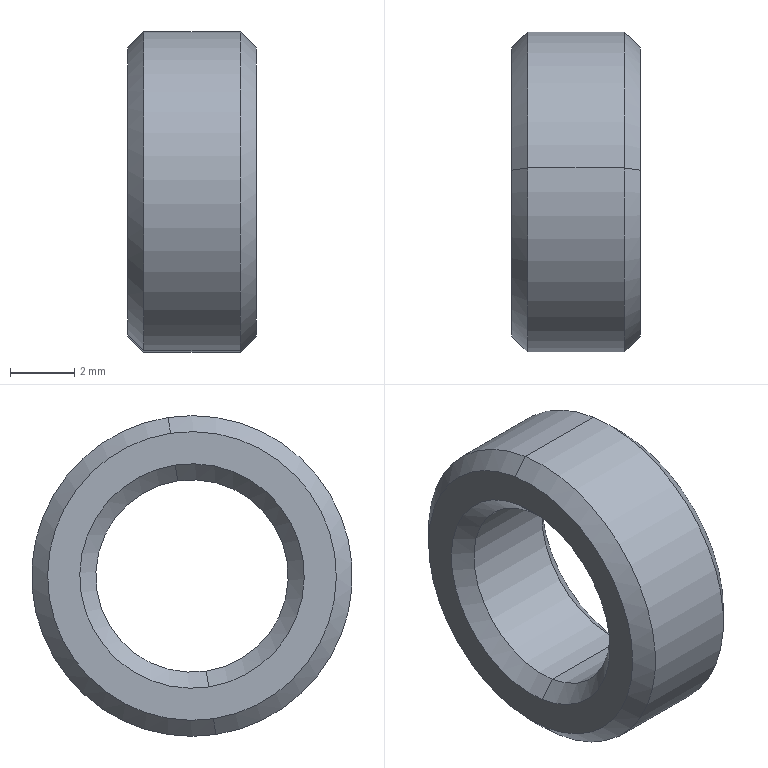Component | SolidWorks | STB-08-000-3-1_STB-08-026-2 | 1 solid | 14 faces | box 4 x 10 x 10 mm | volume 188 mm3 | cone 8 | cylinder 4 | plane 2 | commonest cylinder face diameters 6 x2 10 x2
build123d program:
from build123d import *

# Parameters (mm, degrees)
SKETCH1_R           = 5
BOSS_EXTRUDE1_DEPTH = 2
CUT_EXTRUDE1_REACH  = 10.124
SKETCH2_R           = 3
CHAMFER1_SIZE       = 0.5


with BuildPart() as part:
    # Sketch1 → Boss-Extrude1 (new, symmetric)
    with BuildSketch(Plane(origin=(0, 0, 0), x_dir=(0, 0, -1), z_dir=(1, 0, 0))):
        Circle(SKETCH1_R)
    extrude(amount=BOSS_EXTRUDE1_DEPTH, both=True)

    # Sketch2 → Cut-Extrude1 (cut, up to next)
    with BuildSketch(Plane(origin=(2, 0, 0), x_dir=(0, 0, -1), z_dir=(1, 0, 0)), mode=Mode.PRIVATE) as cut_extrude1_sk1:
        Circle(SKETCH2_R)
    cut_extrude1_tool1 = extrude(cut_extrude1_sk1.sketch, amount=-CUT_EXTRUDE1_REACH, mode=Mode.PRIVATE) & part.part
    add(cut_extrude1_tool1.solids().sort_by_distance((2, 0, 0))[0], mode=Mode.SUBTRACT)

    # Chamfer1
    chamfer1_edges = [part.edges().sort_by_distance(p)[0] for p in [
        (-2, 0, 5),
        (2, 0, 5),
        (2, 0, 3),
        (-2, 0, 3),
    ]]
    chamfer(chamfer1_edges, length=CHAMFER1_SIZE)


solid = part.part

# Placed as in the assembly
solid = solid.moved(Location((-221.904, 437.999, -10), (0, 0, 0)))
STEP:
#1=COLOUR_RGB('',0.7922,0.8196,0.9333);
#2=FILL_AREA_STYLE_COLOUR('',#1);
#3=FILL_AREA_STYLE('',(#2));
#4=SURFACE_STYLE_FILL_AREA(#3);
#5=SURFACE_SIDE_STYLE('',(#4));
#6=SURFACE_STYLE_USAGE(.BOTH.,#5);
#7=PRESENTATION_STYLE_ASSIGNMENT((#6));
#8=CARTESIAN_POINT('',(-8.658,17.218,-0.5689));
#9=VERTEX_POINT('',#8);
#10=CARTESIAN_POINT('',(-8.658,17.27,-0.2185));
#11=VERTEX_POINT('',#10);
#12=CARTESIAN_POINT('',(-8.658,17.244,-0.3937));
#13=DIRECTION('',(1.,0.,0.));
#14=DIRECTION('',(0.,-0.1487,-0.9889));
#15=AXIS2_PLACEMENT_3D('',#12,#13,#14);
#16=CIRCLE('',#15,0.1772);
#17=EDGE_CURVE('',#9,#11,#16,.T.);
#18=ORIENTED_EDGE('',*,*,#17,.F.);
#19=CARTESIAN_POINT('',(-8.677,17.215,-0.5884));
#20=VERTEX_POINT('',#19);
#21=CARTESIAN_POINT('',(-8.658,17.218,-0.5689));
#22=DIRECTION('',(-0.7071,-0.1051,-0.6992));
#23=VECTOR('',#22,39.37);
#24=LINE('',#21,#23);
#25=EDGE_CURVE('',#9,#20,#24,.T.);
#26=ORIENTED_EDGE('',*,*,#25,.T.);
#27=CARTESIAN_POINT('',(-8.677,17.273,-0.199));
#28=VERTEX_POINT('',#27);
#29=CARTESIAN_POINT('',(-8.677,17.244,-0.3937));
#30=DIRECTION('',(-1.,0.,0.));
#31=DIRECTION('',(0.,-0.1487,-0.9889));
#32=AXIS2_PLACEMENT_3D('',#29,#30,#31);
#33=CIRCLE('',#32,0.1969);
#34=EDGE_CURVE('',#28,#20,#33,.T.);
#35=ORIENTED_EDGE('',*,*,#34,.F.);
#36=CARTESIAN_POINT('',(-8.658,17.27,-0.2185));
#37=DIRECTION('',(-0.7071,0.1051,0.6992));
#38=VECTOR('',#37,39.37);
#39=LINE('',#36,#38);
#40=EDGE_CURVE('',#11,#28,#39,.T.);
#41=ORIENTED_EDGE('',*,*,#40,.F.);
#42=EDGE_LOOP('',(#18,#26,#35,#41));
#43=FACE_OUTER_BOUND('',#42,.T.);
#44=CARTESIAN_POINT('',(-8.658,17.244,-0.3937));
#45=DIRECTION('',(-1.,0.,0.));
#46=DIRECTION('',(0.,0.1487,0.9889));
#47=AXIS2_PLACEMENT_3D('',#44,#45,#46);
#48=CONICAL_SURFACE('',#47,0.1772,0.7854);
#49=ADVANCED_FACE('',(#43),#48,.T.);
#50=CARTESIAN_POINT('',(-8.677,17.262,-0.2769));
#51=VERTEX_POINT('',#50);
#52=CARTESIAN_POINT('',(-8.677,17.226,-0.5105));
#53=VERTEX_POINT('',#52);
#54=CARTESIAN_POINT('',(-8.677,17.244,-0.3937));
#55=DIRECTION('',(1.,0.,0.));
#56=DIRECTION('',(0.,-0.1487,-0.9889));
#57=AXIS2_PLACEMENT_3D('',#54,#55,#56);
#58=CIRCLE('',#57,0.1181);
#59=EDGE_CURVE('',#51,#53,#58,.T.);
#60=ORIENTED_EDGE('',*,*,#59,.F.);
#61=CARTESIAN_POINT('',(-8.658,17.265,-0.2574));
#62=VERTEX_POINT('',#61);
#63=CARTESIAN_POINT('',(-8.677,17.262,-0.2769));
#64=DIRECTION('',(0.7071,0.1051,0.6992));
#65=VECTOR('',#64,39.37);
#66=LINE('',#63,#65);
#67=EDGE_CURVE('',#51,#62,#66,.T.);
#68=ORIENTED_EDGE('',*,*,#67,.T.);
#69=CARTESIAN_POINT('',(-8.658,17.224,-0.53));
#70=VERTEX_POINT('',#69);
#71=CARTESIAN_POINT('',(-8.658,17.244,-0.3937));
#72=DIRECTION('',(-1.,0.,0.));
#73=DIRECTION('',(0.,-0.1487,-0.9889));
#74=AXIS2_PLACEMENT_3D('',#71,#72,#73);
#75=CIRCLE('',#74,0.1378);
#76=EDGE_CURVE('',#70,#62,#75,.T.);
#77=ORIENTED_EDGE('',*,*,#76,.F.);
#78=CARTESIAN_POINT('',(-8.677,17.226,-0.5105));
#79=DIRECTION('',(0.7071,-0.1051,-0.6992));
#80=VECTOR('',#79,39.37);
#81=LINE('',#78,#80);
#82=EDGE_CURVE('',#53,#70,#81,.T.);
#83=ORIENTED_EDGE('',*,*,#82,.F.);
#84=EDGE_LOOP('',(#60,#68,#77,#83));
#85=FACE_OUTER_BOUND('',#84,.T.);
#86=CARTESIAN_POINT('',(-8.677,17.244,-0.3937));
#87=DIRECTION('',(1.,0.,0.));
#88=DIRECTION('',(0.,-0.1487,-0.9889));
#89=AXIS2_PLACEMENT_3D('',#86,#87,#88);
#90=CONICAL_SURFACE('',#89,0.1181,0.7854);
#91=ADVANCED_FACE('',(#85),#90,.F.);
#92=CARTESIAN_POINT('',(-8.795,17.226,-0.5105));
#93=VERTEX_POINT('',#92);
#94=CARTESIAN_POINT('',(-8.795,17.262,-0.2769));
#95=VERTEX_POINT('',#94);
#96=CARTESIAN_POINT('',(-8.795,17.244,-0.3937));
#97=DIRECTION('',(-1.,0.,0.));
#98=DIRECTION('',(0.,-0.1487,-0.9889));
#99=AXIS2_PLACEMENT_3D('',#96,#97,#98);
#100=CIRCLE('',#99,0.1181);
#101=EDGE_CURVE('',#93,#95,#100,.T.);
#102=ORIENTED_EDGE('',*,*,#101,.F.);
#103=CARTESIAN_POINT('',(-8.815,17.224,-0.53));
#104=VERTEX_POINT('',#103);
#105=CARTESIAN_POINT('',(-8.795,17.226,-0.5105));
#106=DIRECTION('',(-0.7071,-0.1051,-0.6992));
#107=VECTOR('',#106,39.37);
#108=LINE('',#105,#107);
#109=EDGE_CURVE('',#93,#104,#108,.T.);
#110=ORIENTED_EDGE('',*,*,#109,.T.);
#111=CARTESIAN_POINT('',(-8.815,17.265,-0.2574));
#112=VERTEX_POINT('',#111);
#113=CARTESIAN_POINT('',(-8.815,17.244,-0.3937));
#114=DIRECTION('',(1.,0.,0.));
#115=DIRECTION('',(0.,-0.1487,-0.9889));
#116=AXIS2_PLACEMENT_3D('',#113,#114,#115);
#117=CIRCLE('',#116,0.1378);
#118=EDGE_CURVE('',#112,#104,#117,.T.);
#119=ORIENTED_EDGE('',*,*,#118,.F.);
#120=CARTESIAN_POINT('',(-8.795,17.262,-0.2769));
#121=DIRECTION('',(-0.7071,0.1051,0.6992));
#122=VECTOR('',#121,39.37);
#123=LINE('',#120,#122);
#124=EDGE_CURVE('',#95,#112,#123,.T.);
#125=ORIENTED_EDGE('',*,*,#124,.F.);
#126=EDGE_LOOP('',(#102,#110,#119,#125));
#127=FACE_OUTER_BOUND('',#126,.T.);
#128=CARTESIAN_POINT('',(-8.795,17.244,-0.3937));
#129=DIRECTION('',(-1.,0.,0.));
#130=DIRECTION('',(0.,0.1487,0.9889));
#131=AXIS2_PLACEMENT_3D('',#128,#129,#130);
#132=CONICAL_SURFACE('',#131,0.1181,0.7854);
#133=ADVANCED_FACE('',(#127),#132,.F.);
#134=CARTESIAN_POINT('',(-8.815,17.27,-0.2185));
#135=VERTEX_POINT('',#134);
#136=CARTESIAN_POINT('',(-8.815,17.218,-0.5689));
#137=VERTEX_POINT('',#136);
#138=CARTESIAN_POINT('',(-8.815,17.244,-0.3937));
#139=DIRECTION('',(-1.,0.,0.));
#140=DIRECTION('',(0.,-0.1487,-0.9889));
#141=AXIS2_PLACEMENT_3D('',#138,#139,#140);
#142=CIRCLE('',#141,0.1772);
#143=EDGE_CURVE('',#135,#137,#142,.T.);
#144=ORIENTED_EDGE('',*,*,#143,.F.);
#145=CARTESIAN_POINT('',(-8.795,17.273,-0.199));
#146=VERTEX_POINT('',#145);
#147=CARTESIAN_POINT('',(-8.795,17.273,-0.199));
#148=DIRECTION('',(0.7071,0.1051,0.6992));
#149=VECTOR('',#148,39.37);
#150=LINE('',#147,#149);
#151=EDGE_CURVE('',#135,#146,#150,.T.);
#152=ORIENTED_EDGE('',*,*,#151,.T.);
#153=CARTESIAN_POINT('',(-8.795,17.215,-0.5884));
#154=VERTEX_POINT('',#153);
#155=CARTESIAN_POINT('',(-8.795,17.244,-0.3937));
#156=DIRECTION('',(1.,0.,0.));
#157=DIRECTION('',(0.,-0.1487,-0.9889));
#158=AXIS2_PLACEMENT_3D('',#155,#156,#157);
#159=CIRCLE('',#158,0.1969);
#160=EDGE_CURVE('',#154,#146,#159,.T.);
#161=ORIENTED_EDGE('',*,*,#160,.F.);
#162=CARTESIAN_POINT('',(-8.795,17.215,-0.5884));
#163=DIRECTION('',(0.7071,-0.1051,-0.6992));
#164=VECTOR('',#163,39.37);
#165=LINE('',#162,#164);
#166=EDGE_CURVE('',#137,#154,#165,.T.);
#167=ORIENTED_EDGE('',*,*,#166,.F.);
#168=EDGE_LOOP('',(#144,#152,#161,#167));
#169=FACE_OUTER_BOUND('',#168,.T.);
#170=CARTESIAN_POINT('',(-8.795,17.244,-0.3937));
#171=DIRECTION('',(1.,0.,0.));
#172=DIRECTION('',(0.,-0.1487,-0.9889));
#173=AXIS2_PLACEMENT_3D('',#170,#171,#172);
#174=CONICAL_SURFACE('',#173,0.1969,0.7854);
#175=ADVANCED_FACE('',(#169),#174,.T.);
#176=ORIENTED_EDGE('',*,*,#101,.T.);
#177=CARTESIAN_POINT('',(-8.815,17.262,-0.2769));
#178=DIRECTION('',(1.,0.,0.));
#179=VECTOR('',#178,39.37);
#180=LINE('',#177,#179);
#181=EDGE_CURVE('',#95,#51,#180,.T.);
#182=ORIENTED_EDGE('',*,*,#181,.T.);
#183=ORIENTED_EDGE('',*,*,#59,.T.);
#184=CARTESIAN_POINT('',(-8.815,17.226,-0.5105));
#185=DIRECTION('',(1.,0.,0.));
#186=VECTOR('',#185,39.37);
#187=LINE('',#184,#186);
#188=EDGE_CURVE('',#93,#53,#187,.T.);
#189=ORIENTED_EDGE('',*,*,#188,.F.);
#190=EDGE_LOOP('',(#176,#182,#183,#189));
#191=FACE_OUTER_BOUND('',#190,.T.);
#192=CARTESIAN_POINT('',(-8.815,17.244,-0.3937));
#193=DIRECTION('',(1.,0.,0.));
#194=DIRECTION('',(0.,-0.1487,-0.9889));
#195=AXIS2_PLACEMENT_3D('',#192,#193,#194);
#196=CYLINDRICAL_SURFACE('',#195,0.1181);
#197=ADVANCED_FACE('',(#191),#196,.F.);
#198=ORIENTED_EDGE('',*,*,#34,.T.);
#199=CARTESIAN_POINT('',(-8.658,17.215,-0.5884));
#200=DIRECTION('',(-1.,0.,0.));
#201=VECTOR('',#200,39.37);
#202=LINE('',#199,#201);
#203=EDGE_CURVE('',#20,#154,#202,.T.);
#204=ORIENTED_EDGE('',*,*,#203,.T.);
#205=ORIENTED_EDGE('',*,*,#160,.T.);
#206=CARTESIAN_POINT('',(-8.658,17.273,-0.199));
#207=DIRECTION('',(-1.,0.,0.));
#208=VECTOR('',#207,39.37);
#209=LINE('',#206,#208);
#210=EDGE_CURVE('',#28,#146,#209,.T.);
#211=ORIENTED_EDGE('',*,*,#210,.F.);
#212=EDGE_LOOP('',(#198,#204,#205,#211));
#213=FACE_OUTER_BOUND('',#212,.T.);
#214=CARTESIAN_POINT('',(-8.658,17.244,-0.3937));
#215=DIRECTION('',(-1.,0.,0.));
#216=DIRECTION('',(0.,0.1487,0.9889));
#217=AXIS2_PLACEMENT_3D('',#214,#215,#216);
#218=CYLINDRICAL_SURFACE('',#217,0.1969);
#219=ADVANCED_FACE('',(#213),#218,.T.);
#220=ORIENTED_EDGE('',*,*,#203,.F.);
#221=CARTESIAN_POINT('',(-8.677,17.244,-0.3937));
#222=DIRECTION('',(-1.,0.,0.));
#223=DIRECTION('',(0.,-0.1487,-0.9889));
#224=AXIS2_PLACEMENT_3D('',#221,#222,#223);
#225=CIRCLE('',#224,0.1969);
#226=EDGE_CURVE('',#20,#28,#225,.T.);
#227=ORIENTED_EDGE('',*,*,#226,.T.);
#228=ORIENTED_EDGE('',*,*,#210,.T.);
#229=CARTESIAN_POINT('',(-8.795,17.244,-0.3937));
#230=DIRECTION('',(1.,0.,0.));
#231=DIRECTION('',(0.,-0.1487,-0.9889));
#232=AXIS2_PLACEMENT_3D('',#229,#230,#231);
#233=CIRCLE('',#232,0.1969);
#234=EDGE_CURVE('',#146,#154,#233,.T.);
#235=ORIENTED_EDGE('',*,*,#234,.T.);
#236=EDGE_LOOP('',(#220,#227,#228,#235));
#237=FACE_OUTER_BOUND('',#236,.T.);
#238=CARTESIAN_POINT('',(-8.658,17.244,-0.3937));
#239=DIRECTION('',(-1.,0.,0.));
#240=DIRECTION('',(0.,0.1487,0.9889));
#241=AXIS2_PLACEMENT_3D('',#238,#239,#240);
#242=CYLINDRICAL_SURFACE('',#241,0.1969);
#243=ADVANCED_FACE('',(#237),#242,.T.);
#244=ORIENTED_EDGE('',*,*,#76,.T.);
#245=CARTESIAN_POINT('',(-8.658,17.244,-0.3937));
#246=DIRECTION('',(-1.,0.,0.));
#247=DIRECTION('',(0.,-0.1487,-0.9889));
#248=AXIS2_PLACEMENT_3D('',#245,#246,#247);
#249=CIRCLE('',#248,0.1378);
#250=EDGE_CURVE('',#62,#70,#249,.T.);
#251=ORIENTED_EDGE('',*,*,#250,.T.);
#252=EDGE_LOOP('',(#244,#251));
#253=FACE_BOUND('',#252,.T.);
#254=CARTESIAN_POINT('',(-8.658,17.244,-0.3937));
#255=DIRECTION('',(1.,0.,0.));
#256=DIRECTION('',(0.,-0.1487,-0.9889));
#257=AXIS2_PLACEMENT_3D('',#254,#255,#256);
#258=CIRCLE('',#257,0.1772);
#259=EDGE_CURVE('',#11,#9,#258,.T.);
#260=ORIENTED_EDGE('',*,*,#259,.T.);
#261=ORIENTED_EDGE('',*,*,#17,.T.);
#262=EDGE_LOOP('',(#260,#261));
#263=FACE_OUTER_BOUND('',#262,.T.);
#264=CARTESIAN_POINT('',(-8.658,17.244,-0.3937));
#265=DIRECTION('',(1.,0.,0.));
#266=DIRECTION('',(0.,-0.1487,-0.9889));
#267=AXIS2_PLACEMENT_3D('',#264,#265,#266);
#268=PLANE('',#267);
#269=ADVANCED_FACE('',(#253,#263),#268,.T.);
#270=CARTESIAN_POINT('',(-8.815,17.244,-0.3937));
#271=DIRECTION('',(-1.,0.,0.));
#272=DIRECTION('',(0.,-0.1487,-0.9889));
#273=AXIS2_PLACEMENT_3D('',#270,#271,#272);
#274=CIRCLE('',#273,0.1772);
#275=EDGE_CURVE('',#137,#135,#274,.T.);
#276=ORIENTED_EDGE('',*,*,#275,.T.);
#277=ORIENTED_EDGE('',*,*,#143,.T.);
#278=EDGE_LOOP('',(#276,#277));
#279=FACE_OUTER_BOUND('',#278,.T.);
#280=ORIENTED_EDGE('',*,*,#118,.T.);
#281=CARTESIAN_POINT('',(-8.815,17.244,-0.3937));
#282=DIRECTION('',(1.,0.,0.));
#283=DIRECTION('',(0.,-0.1487,-0.9889));
#284=AXIS2_PLACEMENT_3D('',#281,#282,#283);
#285=CIRCLE('',#284,0.1378);
#286=EDGE_CURVE('',#104,#112,#285,.T.);
#287=ORIENTED_EDGE('',*,*,#286,.T.);
#288=EDGE_LOOP('',(#280,#287));
#289=FACE_BOUND('',#288,.T.);
#290=CARTESIAN_POINT('',(-8.815,17.244,-0.3937));
#291=DIRECTION('',(1.,0.,0.));
#292=DIRECTION('',(0.,-0.1487,-0.9889));
#293=AXIS2_PLACEMENT_3D('',#290,#291,#292);
#294=PLANE('',#293);
#295=ADVANCED_FACE('',(#279,#289),#294,.F.);
#296=ORIENTED_EDGE('',*,*,#181,.F.);
#297=CARTESIAN_POINT('',(-8.795,17.244,-0.3937));
#298=DIRECTION('',(-1.,0.,0.));
#299=DIRECTION('',(0.,-0.1487,-0.9889));
#300=AXIS2_PLACEMENT_3D('',#297,#298,#299);
#301=CIRCLE('',#300,0.1181);
#302=EDGE_CURVE('',#95,#93,#301,.T.);
#303=ORIENTED_EDGE('',*,*,#302,.T.);
#304=ORIENTED_EDGE('',*,*,#188,.T.);
#305=CARTESIAN_POINT('',(-8.677,17.244,-0.3937));
#306=DIRECTION('',(1.,0.,0.));
#307=DIRECTION('',(0.,-0.1487,-0.9889));
#308=AXIS2_PLACEMENT_3D('',#305,#306,#307);
#309=CIRCLE('',#308,0.1181);
#310=EDGE_CURVE('',#53,#51,#309,.T.);
#311=ORIENTED_EDGE('',*,*,#310,.T.);
#312=EDGE_LOOP('',(#296,#303,#304,#311));
#313=FACE_OUTER_BOUND('',#312,.T.);
#314=CARTESIAN_POINT('',(-8.815,17.244,-0.3937));
#315=DIRECTION('',(1.,0.,0.));
#316=DIRECTION('',(0.,-0.1487,-0.9889));
#317=AXIS2_PLACEMENT_3D('',#314,#315,#316);
#318=CYLINDRICAL_SURFACE('',#317,0.1181);
#319=ADVANCED_FACE('',(#313),#318,.F.);
#320=ORIENTED_EDGE('',*,*,#151,.F.);
#321=ORIENTED_EDGE('',*,*,#275,.F.);
#322=ORIENTED_EDGE('',*,*,#166,.T.);
#323=ORIENTED_EDGE('',*,*,#234,.F.);
#324=EDGE_LOOP('',(#320,#321,#322,#323));
#325=FACE_OUTER_BOUND('',#324,.T.);
#326=CARTESIAN_POINT('',(-8.795,17.244,-0.3937));
#327=DIRECTION('',(1.,0.,0.));
#328=DIRECTION('',(0.,-0.1487,-0.9889));
#329=AXIS2_PLACEMENT_3D('',#326,#327,#328);
#330=CONICAL_SURFACE('',#329,0.1969,0.7854);
#331=ADVANCED_FACE('',(#325),#330,.T.);
#332=ORIENTED_EDGE('',*,*,#109,.F.);
#333=ORIENTED_EDGE('',*,*,#302,.F.);
#334=ORIENTED_EDGE('',*,*,#124,.T.);
#335=ORIENTED_EDGE('',*,*,#286,.F.);
#336=EDGE_LOOP('',(#332,#333,#334,#335));
#337=FACE_OUTER_BOUND('',#336,.T.);
#338=CARTESIAN_POINT('',(-8.795,17.244,-0.3937));
#339=DIRECTION('',(-1.,0.,0.));
#340=DIRECTION('',(0.,0.1487,0.9889));
#341=AXIS2_PLACEMENT_3D('',#338,#339,#340);
#342=CONICAL_SURFACE('',#341,0.1181,0.7854);
#343=ADVANCED_FACE('',(#337),#342,.F.);
#344=ORIENTED_EDGE('',*,*,#67,.F.);
#345=ORIENTED_EDGE('',*,*,#310,.F.);
#346=ORIENTED_EDGE('',*,*,#82,.T.);
#347=ORIENTED_EDGE('',*,*,#250,.F.);
#348=EDGE_LOOP('',(#344,#345,#346,#347));
#349=FACE_OUTER_BOUND('',#348,.T.);
#350=CARTESIAN_POINT('',(-8.677,17.244,-0.3937));
#351=DIRECTION('',(1.,0.,0.));
#352=DIRECTION('',(0.,-0.1487,-0.9889));
#353=AXIS2_PLACEMENT_3D('',#350,#351,#352);
#354=CONICAL_SURFACE('',#353,0.1181,0.7854);
#355=ADVANCED_FACE('',(#349),#354,.F.);
#356=ORIENTED_EDGE('',*,*,#25,.F.);
#357=ORIENTED_EDGE('',*,*,#259,.F.);
#358=ORIENTED_EDGE('',*,*,#40,.T.);
#359=ORIENTED_EDGE('',*,*,#226,.F.);
#360=EDGE_LOOP('',(#356,#357,#358,#359));
#361=FACE_OUTER_BOUND('',#360,.T.);
#362=CARTESIAN_POINT('',(-8.658,17.244,-0.3937));
#363=DIRECTION('',(-1.,0.,0.));
#364=DIRECTION('',(0.,0.1487,0.9889));
#365=AXIS2_PLACEMENT_3D('',#362,#363,#364);
#366=CONICAL_SURFACE('',#365,0.1772,0.7854);
#367=ADVANCED_FACE('',(#361),#366,.T.);
#368=CLOSED_SHELL('',(#49,#91,#133,#175,#197,#219,#243,#269,#295,#319,#331,#343,#355,#367));
#369=MANIFOLD_SOLID_BREP('',#368);
#370=STYLED_ITEM('',(#7),#369);
#371=(LENGTH_UNIT()NAMED_UNIT(*)SI_UNIT($,.METRE.));
#372=LENGTH_MEASURE_WITH_UNIT(LENGTH_MEASURE(0.0254),#371);
#373=DIMENSIONAL_EXPONENTS(1.,0.,0.,0.,0.,0.,0.);
#374=(CONVERSION_BASED_UNIT('',#372)LENGTH_UNIT()NAMED_UNIT(#373));
#375=UNCERTAINTY_MEASURE_WITH_UNIT(LENGTH_MEASURE(0.00001),#374,'','');
#376=(NAMED_UNIT(*)PLANE_ANGLE_UNIT()SI_UNIT($,.RADIAN.));
#377=(NAMED_UNIT(*)SI_UNIT($,.STERADIAN.)SOLID_ANGLE_UNIT());
#378=(GEOMETRIC_REPRESENTATION_CONTEXT(3)GLOBAL_UNCERTAINTY_ASSIGNED_CONTEXT((#375))GLOBAL_UNIT_ASSIGNED_CONTEXT((#374,#376,#377))REPRESENTATION_CONTEXT('',''));
#379=MECHANICAL_DESIGN_GEOMETRIC_PRESENTATION_REPRESENTATION('',(#370),#378);
#380=CARTESIAN_POINT('',(0.,0.,0.));
#381=DIRECTION('',(0.,0.,1.));
#382=DIRECTION('',(1.,0.,0.));
#383=AXIS2_PLACEMENT_3D('',#380,#381,#382);
#384=(LENGTH_UNIT()NAMED_UNIT(*)SI_UNIT($,.METRE.));
#385=LENGTH_MEASURE_WITH_UNIT(LENGTH_MEASURE(0.0254),#384);
#386=DIMENSIONAL_EXPONENTS(1.,0.,0.,0.,0.,0.,0.);
#387=(CONVERSION_BASED_UNIT('',#385)LENGTH_UNIT()NAMED_UNIT(#386));
#388=UNCERTAINTY_MEASURE_WITH_UNIT(LENGTH_MEASURE(0.00001),#387,'','');
#389=(NAMED_UNIT(*)PLANE_ANGLE_UNIT()SI_UNIT($,.RADIAN.));
#390=(NAMED_UNIT(*)SI_UNIT($,.STERADIAN.)SOLID_ANGLE_UNIT());
#391=(GEOMETRIC_REPRESENTATION_CONTEXT(3)GLOBAL_UNCERTAINTY_ASSIGNED_CONTEXT((#388))GLOBAL_UNIT_ASSIGNED_CONTEXT((#387,#389,#390))REPRESENTATION_CONTEXT('',''));
#392=ADVANCED_BREP_SHAPE_REPRESENTATION('',(#369,#383),#391);
#393=PRESENTATION_LAYER_ASSIGNMENT('','',(#370));